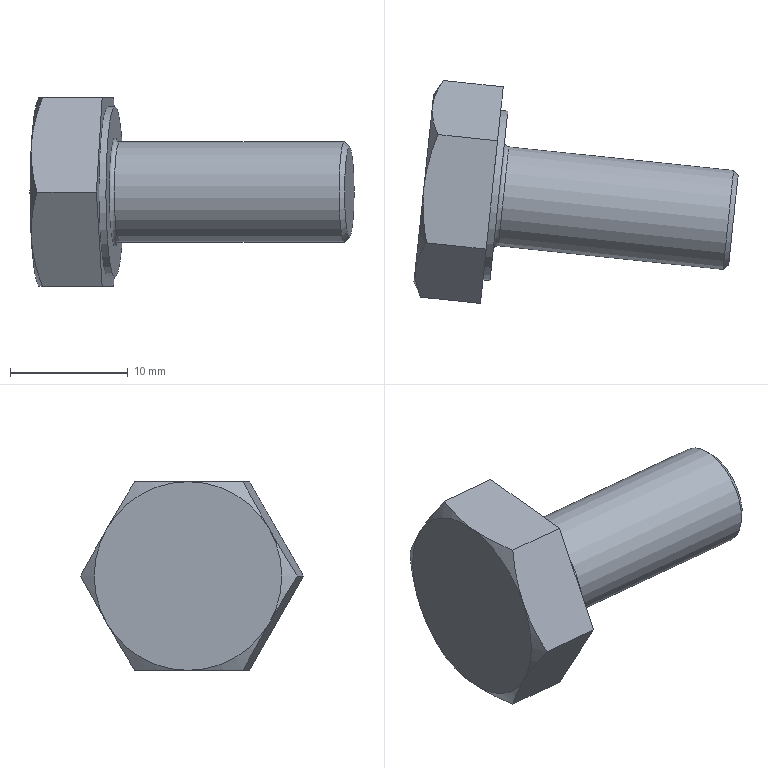Component | NX | GB-T5782-2000_M10X20 | 1 solid | 20 faces | volume 2514 mm3 | plane 10 | cone 7 | cylinder 2 | torus 1 | commonest cylinder face diameters 14.47 x1 8.5 x1